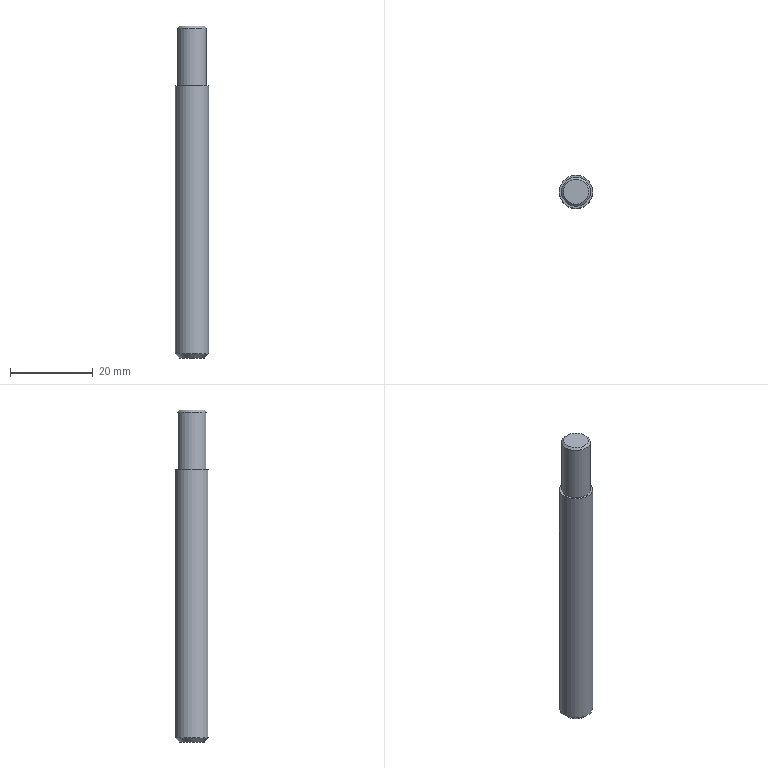Component | NX | LG_ADJ_SUPPORT_2 | 1 solid | 7 faces | box 8 x 8 x 80 mm | volume 3834 mm3 | plane 3 | cylinder 2 | cone 2 | commonest cylinder face diameters 8 x1 6.98 x1
STEP:
#1=CARTESIAN_POINT('',(0.,0.,0.));
#2=DIRECTION('',(0.,0.,1.));
#3=DIRECTION('',(1.,0.,0.));
#4=AXIS2_PLACEMENT_3D('',#1,#2,#3);
#5=CARTESIAN_POINT('',(-91.,-45.,-251.));
#6=VERTEX_POINT('',#5);
#7=CARTESIAN_POINT('',(-88.,-45.,-251.));
#8=DIRECTION('',(0.,0.,-1.));
#9=DIRECTION('',(-1.,0.,0.));
#10=AXIS2_PLACEMENT_3D('',#7,#8,#9);
#11=CIRCLE('',#10,3.);
#12=CARTESIAN_POINT('',(-88.,-45.,-251.));
#13=DIRECTION('',(0.,0.,-1.));
#14=DIRECTION('',(-1.,0.,0.));
#15=AXIS2_PLACEMENT_3D('',#12,#13,#14);
#16=PLANE('',#15);
#17=CARTESIAN_POINT('',(0.,0.));
#18=DIRECTION('',(1.,0.));
#19=AXIS2_PLACEMENT_2D('',#17,#18);
#20=CIRCLE('',#19,3.);
#21=(GEOMETRIC_REPRESENTATION_CONTEXT(2)PARAMETRIC_REPRESENTATION_CONTEXT()REPRESENTATION_CONTEXT('',''));
#22=DEFINITIONAL_REPRESENTATION('',(#20),#21);
#23=PCURVE('',#16,#22);
#24=CARTESIAN_POINT('',(-88.,-45.,-250.));
#25=DIRECTION('',(0.,0.,1.));
#26=DIRECTION('',(1.,0.,0.));
#27=AXIS2_PLACEMENT_3D('',#24,#25,#26);
#28=CONICAL_SURFACE('',#27,4.,0.7854);
#29=CARTESIAN_POINT('',(9.425,-1.));
#30=DIRECTION('',(-1.,0.));
#31=VECTOR('',#30,1.);
#32=LINE('',#29,#31);
#33=(GEOMETRIC_REPRESENTATION_CONTEXT(2)PARAMETRIC_REPRESENTATION_CONTEXT()REPRESENTATION_CONTEXT('',''));
#34=DEFINITIONAL_REPRESENTATION('',(#32),#33);
#35=PCURVE('',#28,#34);
#36=SURFACE_CURVE('',#11,(#23,#35),.PCURVE_S1.);
#37=EDGE_CURVE('',#6,#6,#36,.T.);
#38=ORIENTED_EDGE('',*,*,#37,.T.);
#39=EDGE_LOOP('',(#38));
#40=FACE_BOUND('',#39,.T.);
#41=ADVANCED_FACE('',(#40),#16,.T.);
#42=CARTESIAN_POINT('',(-92.,-45.,-185.4));
#43=VERTEX_POINT('',#42);
#44=CARTESIAN_POINT('',(-88.,-45.,-185.4));
#45=DIRECTION('',(0.,0.,1.));
#46=DIRECTION('',(-1.,0.,0.));
#47=AXIS2_PLACEMENT_3D('',#44,#45,#46);
#48=CIRCLE('',#47,4.);
#49=CARTESIAN_POINT('',(-88.,-45.,-251.));
#50=DIRECTION('',(0.,0.,1.));
#51=DIRECTION('',(1.,0.,0.));
#52=AXIS2_PLACEMENT_3D('',#49,#50,#51);
#53=CYLINDRICAL_SURFACE('',#52,4.);
#54=CARTESIAN_POINT('',(3.142,65.6));
#55=DIRECTION('',(1.,0.));
#56=VECTOR('',#55,1.);
#57=LINE('',#54,#56);
#58=(GEOMETRIC_REPRESENTATION_CONTEXT(2)PARAMETRIC_REPRESENTATION_CONTEXT()REPRESENTATION_CONTEXT('',''));
#59=DEFINITIONAL_REPRESENTATION('',(#57),#58);
#60=PCURVE('',#53,#59);
#61=CARTESIAN_POINT('',(-88.,-45.,-185.4));
#62=DIRECTION('',(0.,0.,-1.));
#63=DIRECTION('',(-1.,0.,0.));
#64=AXIS2_PLACEMENT_3D('',#61,#62,#63);
#65=PLANE('',#64);
#66=CARTESIAN_POINT('',(4.,0.));
#67=CARTESIAN_POINT('',(4.,-6.928));
#68=CARTESIAN_POINT('',(-2.,-3.464));
#69=CARTESIAN_POINT('',(-8.,-0.));
#70=CARTESIAN_POINT('',(-2.,3.464));
#71=CARTESIAN_POINT('',(4.,6.928));
#72=CARTESIAN_POINT('',(4.,0.));
#73=(BOUNDED_CURVE()B_SPLINE_CURVE(2,(#66,#67,#68,#69,#70,#71,#72),.UNSPECIFIED.,.T.,.F.)B_SPLINE_CURVE_WITH_KNOTS((1,2,2,2,2,1),(-2.094,0.,2.094,4.189,6.283,8.378),.UNSPECIFIED.)CURVE()GEOMETRIC_REPRESENTATION_ITEM()RATIONAL_B_SPLINE_CURVE((1.,0.5,1.,0.5,1.,0.5,1.))REPRESENTATION_ITEM(''));
#74=(GEOMETRIC_REPRESENTATION_CONTEXT(2)PARAMETRIC_REPRESENTATION_CONTEXT()REPRESENTATION_CONTEXT('',''));
#75=DEFINITIONAL_REPRESENTATION('',(#73),#74);
#76=PCURVE('',#65,#75);
#77=SURFACE_CURVE('',#48,(#60,#76),.PCURVE_S1.);
#78=EDGE_CURVE('',#43,#43,#77,.T.);
#79=ORIENTED_EDGE('',*,*,#78,.F.);
#80=CARTESIAN_POINT('',(-92.,-45.,-250.));
#81=VERTEX_POINT('',#80);
#82=CARTESIAN_POINT('',(-92.,-45.,-250.));
#83=CARTESIAN_POINT('',(-92.,-45.,-185.4));
#84=B_SPLINE_CURVE_WITH_KNOTS('',1,(#82,#83),.UNSPECIFIED.,.F.,.F.,(2,2),(1.,65.6),.PIECEWISE_BEZIER_KNOTS.);
#85=CARTESIAN_POINT('',(3.142,0.));
#86=DIRECTION('',(0.,1.));
#87=VECTOR('',#86,1.);
#88=LINE('',#85,#87);
#89=(GEOMETRIC_REPRESENTATION_CONTEXT(2)PARAMETRIC_REPRESENTATION_CONTEXT()REPRESENTATION_CONTEXT('',''));
#90=DEFINITIONAL_REPRESENTATION('',(#88),#89);
#91=PCURVE('',#53,#90);
#92=CARTESIAN_POINT('',(9.425,0.));
#93=DIRECTION('',(0.,1.));
#94=VECTOR('',#93,1.);
#95=LINE('',#92,#94);
#96=(GEOMETRIC_REPRESENTATION_CONTEXT(2)PARAMETRIC_REPRESENTATION_CONTEXT()REPRESENTATION_CONTEXT('',''));
#97=DEFINITIONAL_REPRESENTATION('',(#95),#96);
#98=PCURVE('',#53,#97);
#99=SEAM_CURVE('',#84,(#91,#98),.PCURVE_S1.);
#100=EDGE_CURVE('',#81,#43,#99,.T.);
#101=ORIENTED_EDGE('',*,*,#100,.F.);
#102=CARTESIAN_POINT('',(-88.,-45.,-250.));
#103=DIRECTION('',(0.,0.,1.));
#104=DIRECTION('',(-1.,0.,0.));
#105=AXIS2_PLACEMENT_3D('',#102,#103,#104);
#106=CIRCLE('',#105,4.);
#107=CARTESIAN_POINT('',(3.142,1.));
#108=DIRECTION('',(1.,0.));
#109=VECTOR('',#108,1.);
#110=LINE('',#107,#109);
#111=(GEOMETRIC_REPRESENTATION_CONTEXT(2)PARAMETRIC_REPRESENTATION_CONTEXT()REPRESENTATION_CONTEXT('',''));
#112=DEFINITIONAL_REPRESENTATION('',(#110),#111);
#113=PCURVE('',#53,#112);
#114=CARTESIAN_POINT('',(3.142,0.));
#115=DIRECTION('',(1.,0.));
#116=VECTOR('',#115,1.);
#117=LINE('',#114,#116);
#118=(GEOMETRIC_REPRESENTATION_CONTEXT(2)PARAMETRIC_REPRESENTATION_CONTEXT()REPRESENTATION_CONTEXT('',''));
#119=DEFINITIONAL_REPRESENTATION('',(#117),#118);
#120=PCURVE('',#28,#119);
#121=SURFACE_CURVE('',#106,(#113,#120),.PCURVE_S1.);
#122=EDGE_CURVE('',#81,#81,#121,.T.);
#123=ORIENTED_EDGE('',*,*,#122,.T.);
#124=ORIENTED_EDGE('',*,*,#100,.T.);
#125=EDGE_LOOP('',(#79,#101,#123,#124));
#126=FACE_BOUND('',#125,.T.);
#127=ADVANCED_FACE('',(#126),#53,.T.);
#128=ORIENTED_EDGE('',*,*,#37,.F.);
#129=CARTESIAN_POINT('',(-91.,-45.,-251.));
#130=CARTESIAN_POINT('',(-92.,-45.,-250.));
#131=B_SPLINE_CURVE_WITH_KNOTS('',1,(#129,#130),.UNSPECIFIED.,.F.,.F.,(2,2),(-1.414,0.),.PIECEWISE_BEZIER_KNOTS.);
#132=CARTESIAN_POINT('',(9.425,0.));
#133=DIRECTION('',(0.,1.));
#134=VECTOR('',#133,1.);
#135=LINE('',#132,#134);
#136=(GEOMETRIC_REPRESENTATION_CONTEXT(2)PARAMETRIC_REPRESENTATION_CONTEXT()REPRESENTATION_CONTEXT('',''));
#137=DEFINITIONAL_REPRESENTATION('',(#135),#136);
#138=PCURVE('',#28,#137);
#139=CARTESIAN_POINT('',(3.142,0.));
#140=DIRECTION('',(0.,1.));
#141=VECTOR('',#140,1.);
#142=LINE('',#139,#141);
#143=(GEOMETRIC_REPRESENTATION_CONTEXT(2)PARAMETRIC_REPRESENTATION_CONTEXT()REPRESENTATION_CONTEXT('',''));
#144=DEFINITIONAL_REPRESENTATION('',(#142),#143);
#145=PCURVE('',#28,#144);
#146=SEAM_CURVE('',#131,(#138,#145),.PCURVE_S1.);
#147=EDGE_CURVE('',#6,#81,#146,.T.);
#148=ORIENTED_EDGE('',*,*,#147,.T.);
#149=ORIENTED_EDGE('',*,*,#122,.F.);
#150=ORIENTED_EDGE('',*,*,#147,.F.);
#151=EDGE_LOOP('',(#128,#148,#149,#150));
#152=FACE_BOUND('',#151,.T.);
#153=ADVANCED_FACE('',(#152),#28,.T.);
#154=ORIENTED_EDGE('',*,*,#78,.T.);
#155=EDGE_LOOP('',(#154));
#156=FACE_BOUND('',#155,.T.);
#157=CARTESIAN_POINT('',(-91.49,-45.,-185.4));
#158=VERTEX_POINT('',#157);
#159=CARTESIAN_POINT('',(-88.,-45.,-185.4));
#160=DIRECTION('',(0.,0.,1.));
#161=DIRECTION('',(-1.,0.,0.));
#162=AXIS2_PLACEMENT_3D('',#159,#160,#161);
#163=CIRCLE('',#162,3.49);
#164=CARTESIAN_POINT('',(3.49,0.));
#165=CARTESIAN_POINT('',(3.49,-6.045));
#166=CARTESIAN_POINT('',(-1.745,-3.022));
#167=CARTESIAN_POINT('',(-6.98,-0.));
#168=CARTESIAN_POINT('',(-1.745,3.022));
#169=CARTESIAN_POINT('',(3.49,6.045));
#170=CARTESIAN_POINT('',(3.49,0.));
#171=(BOUNDED_CURVE()B_SPLINE_CURVE(2,(#164,#165,#166,#167,#168,#169,#170),.UNSPECIFIED.,.T.,.F.)B_SPLINE_CURVE_WITH_KNOTS((1,2,2,2,2,1),(-2.094,0.,2.094,4.189,6.283,8.378),.UNSPECIFIED.)CURVE()GEOMETRIC_REPRESENTATION_ITEM()RATIONAL_B_SPLINE_CURVE((1.,0.5,1.,0.5,1.,0.5,1.))REPRESENTATION_ITEM(''));
#172=(GEOMETRIC_REPRESENTATION_CONTEXT(2)PARAMETRIC_REPRESENTATION_CONTEXT()REPRESENTATION_CONTEXT('',''));
#173=DEFINITIONAL_REPRESENTATION('',(#171),#172);
#174=PCURVE('',#65,#173);
#175=CARTESIAN_POINT('',(-88.,-45.,-186.4));
#176=DIRECTION('',(0.,0.,1.));
#177=DIRECTION('',(1.,0.,0.));
#178=AXIS2_PLACEMENT_3D('',#175,#176,#177);
#179=CYLINDRICAL_SURFACE('',#178,3.49);
#180=CARTESIAN_POINT('',(3.142,1.));
#181=DIRECTION('',(1.,0.));
#182=VECTOR('',#181,1.);
#183=LINE('',#180,#182);
#184=(GEOMETRIC_REPRESENTATION_CONTEXT(2)PARAMETRIC_REPRESENTATION_CONTEXT()REPRESENTATION_CONTEXT('',''));
#185=DEFINITIONAL_REPRESENTATION('',(#183),#184);
#186=PCURVE('',#179,#185);
#187=SURFACE_CURVE('',#163,(#174,#186),.PCURVE_S1.);
#188=EDGE_CURVE('',#158,#158,#187,.T.);
#189=ORIENTED_EDGE('',*,*,#188,.F.);
#190=EDGE_LOOP('',(#189));
#191=FACE_BOUND('',#190,.T.);
#192=ADVANCED_FACE('',(#156,#191),#65,.F.);
#193=CARTESIAN_POINT('',(-91.49,-45.,-171.49));
#194=VERTEX_POINT('',#193);
#195=CARTESIAN_POINT('',(-88.,-45.,-171.49));
#196=DIRECTION('',(0.,0.,1.));
#197=DIRECTION('',(-1.,0.,0.));
#198=AXIS2_PLACEMENT_3D('',#195,#196,#197);
#199=CIRCLE('',#198,3.49);
#200=CARTESIAN_POINT('',(3.142,14.91));
#201=DIRECTION('',(1.,0.));
#202=VECTOR('',#201,1.);
#203=LINE('',#200,#202);
#204=(GEOMETRIC_REPRESENTATION_CONTEXT(2)PARAMETRIC_REPRESENTATION_CONTEXT()REPRESENTATION_CONTEXT('',''));
#205=DEFINITIONAL_REPRESENTATION('',(#203),#204);
#206=PCURVE('',#179,#205);
#207=CARTESIAN_POINT('',(-88.,-45.,-172.));
#208=DIRECTION('',(0.,0.,-1.));
#209=DIRECTION('',(-1.,0.,0.));
#210=AXIS2_PLACEMENT_3D('',#207,#208,#209);
#211=CONICAL_SURFACE('',#210,4.,0.7854);
#212=CARTESIAN_POINT('',(6.283,-0.51));
#213=DIRECTION('',(-1.,0.));
#214=VECTOR('',#213,1.);
#215=LINE('',#212,#214);
#216=(GEOMETRIC_REPRESENTATION_CONTEXT(2)PARAMETRIC_REPRESENTATION_CONTEXT()REPRESENTATION_CONTEXT('',''));
#217=DEFINITIONAL_REPRESENTATION('',(#215),#216);
#218=PCURVE('',#211,#217);
#219=SURFACE_CURVE('',#199,(#206,#218),.PCURVE_S1.);
#220=EDGE_CURVE('',#194,#194,#219,.T.);
#221=ORIENTED_EDGE('',*,*,#220,.F.);
#222=CARTESIAN_POINT('',(-91.49,-45.,-185.4));
#223=CARTESIAN_POINT('',(-91.49,-45.,-171.49));
#224=B_SPLINE_CURVE_WITH_KNOTS('',1,(#222,#223),.UNSPECIFIED.,.F.,.F.,(2,2),(1.,14.91),.PIECEWISE_BEZIER_KNOTS.);
#225=CARTESIAN_POINT('',(3.142,0.));
#226=DIRECTION('',(0.,1.));
#227=VECTOR('',#226,1.);
#228=LINE('',#225,#227);
#229=(GEOMETRIC_REPRESENTATION_CONTEXT(2)PARAMETRIC_REPRESENTATION_CONTEXT()REPRESENTATION_CONTEXT('',''));
#230=DEFINITIONAL_REPRESENTATION('',(#228),#229);
#231=PCURVE('',#179,#230);
#232=CARTESIAN_POINT('',(9.425,0.));
#233=DIRECTION('',(0.,1.));
#234=VECTOR('',#233,1.);
#235=LINE('',#232,#234);
#236=(GEOMETRIC_REPRESENTATION_CONTEXT(2)PARAMETRIC_REPRESENTATION_CONTEXT()REPRESENTATION_CONTEXT('',''));
#237=DEFINITIONAL_REPRESENTATION('',(#235),#236);
#238=PCURVE('',#179,#237);
#239=SEAM_CURVE('',#224,(#231,#238),.PCURVE_S1.);
#240=EDGE_CURVE('',#158,#194,#239,.T.);
#241=ORIENTED_EDGE('',*,*,#240,.F.);
#242=ORIENTED_EDGE('',*,*,#188,.T.);
#243=ORIENTED_EDGE('',*,*,#240,.T.);
#244=EDGE_LOOP('',(#221,#241,#242,#243));
#245=FACE_BOUND('',#244,.T.);
#246=ADVANCED_FACE('',(#245),#179,.T.);
#247=CARTESIAN_POINT('',(-85.,-45.,-171.));
#248=VERTEX_POINT('',#247);
#249=CARTESIAN_POINT('',(-91.,-45.,-171.));
#250=VERTEX_POINT('',#249);
#251=CARTESIAN_POINT('',(-88.,-45.,-171.));
#252=DIRECTION('',(0.,0.,1.));
#253=DIRECTION('',(1.,0.,0.));
#254=AXIS2_PLACEMENT_3D('',#251,#252,#253);
#255=CIRCLE('',#254,3.);
#256=CARTESIAN_POINT('',(-88.,-45.,-171.));
#257=DIRECTION('',(0.,0.,1.));
#258=DIRECTION('',(1.,0.,0.));
#259=AXIS2_PLACEMENT_3D('',#256,#257,#258);
#260=PLANE('',#259);
#261=CARTESIAN_POINT('',(0.,0.));
#262=DIRECTION('',(1.,0.));
#263=AXIS2_PLACEMENT_2D('',#261,#262);
#264=CIRCLE('',#263,3.);
#265=(GEOMETRIC_REPRESENTATION_CONTEXT(2)PARAMETRIC_REPRESENTATION_CONTEXT()REPRESENTATION_CONTEXT('',''));
#266=DEFINITIONAL_REPRESENTATION('',(#264),#265);
#267=PCURVE('',#260,#266);
#268=CARTESIAN_POINT('',(3.142,-1.));
#269=DIRECTION('',(-1.,0.));
#270=VECTOR('',#269,1.);
#271=LINE('',#268,#270);
#272=(GEOMETRIC_REPRESENTATION_CONTEXT(2)PARAMETRIC_REPRESENTATION_CONTEXT()REPRESENTATION_CONTEXT('',''));
#273=DEFINITIONAL_REPRESENTATION('',(#271),#272);
#274=PCURVE('',#211,#273);
#275=SURFACE_CURVE('',#255,(#267,#274),.PCURVE_S1.);
#276=EDGE_CURVE('',#248,#250,#275,.T.);
#277=ORIENTED_EDGE('',*,*,#276,.T.);
#278=CARTESIAN_POINT('',(-88.,-45.,-171.));
#279=DIRECTION('',(0.,0.,1.));
#280=DIRECTION('',(1.,0.,0.));
#281=AXIS2_PLACEMENT_3D('',#278,#279,#280);
#282=CIRCLE('',#281,3.);
#283=CARTESIAN_POINT('',(0.,0.));
#284=DIRECTION('',(1.,0.));
#285=AXIS2_PLACEMENT_2D('',#283,#284);
#286=CIRCLE('',#285,3.);
#287=(GEOMETRIC_REPRESENTATION_CONTEXT(2)PARAMETRIC_REPRESENTATION_CONTEXT()REPRESENTATION_CONTEXT('',''));
#288=DEFINITIONAL_REPRESENTATION('',(#286),#287);
#289=PCURVE('',#260,#288);
#290=CARTESIAN_POINT('',(9.425,-1.));
#291=DIRECTION('',(-1.,0.));
#292=VECTOR('',#291,1.);
#293=LINE('',#290,#292);
#294=(GEOMETRIC_REPRESENTATION_CONTEXT(2)PARAMETRIC_REPRESENTATION_CONTEXT()REPRESENTATION_CONTEXT('',''));
#295=DEFINITIONAL_REPRESENTATION('',(#293),#294);
#296=PCURVE('',#211,#295);
#297=SURFACE_CURVE('',#282,(#289,#296),.PCURVE_S1.);
#298=EDGE_CURVE('',#250,#248,#297,.T.);
#299=ORIENTED_EDGE('',*,*,#298,.T.);
#300=EDGE_LOOP('',(#277,#299));
#301=FACE_BOUND('',#300,.T.);
#302=ADVANCED_FACE('',(#301),#260,.T.);
#303=ORIENTED_EDGE('',*,*,#298,.F.);
#304=CARTESIAN_POINT('',(-91.,-45.,-171.));
#305=CARTESIAN_POINT('',(-91.49,-45.,-171.49));
#306=B_SPLINE_CURVE_WITH_KNOTS('',1,(#304,#305),.UNSPECIFIED.,.F.,.F.,(2,2),(-1.414,-0.7212),.PIECEWISE_BEZIER_KNOTS.);
#307=CARTESIAN_POINT('',(6.283,0.));
#308=DIRECTION('',(0.,1.));
#309=VECTOR('',#308,1.);
#310=LINE('',#307,#309);
#311=(GEOMETRIC_REPRESENTATION_CONTEXT(2)PARAMETRIC_REPRESENTATION_CONTEXT()REPRESENTATION_CONTEXT('',''));
#312=DEFINITIONAL_REPRESENTATION('',(#310),#311);
#313=PCURVE('',#211,#312);
#314=CARTESIAN_POINT('',(0.,0.));
#315=DIRECTION('',(0.,1.));
#316=VECTOR('',#315,1.);
#317=LINE('',#314,#316);
#318=(GEOMETRIC_REPRESENTATION_CONTEXT(2)PARAMETRIC_REPRESENTATION_CONTEXT()REPRESENTATION_CONTEXT('',''));
#319=DEFINITIONAL_REPRESENTATION('',(#317),#318);
#320=PCURVE('',#211,#319);
#321=SEAM_CURVE('',#306,(#313,#320),.PCURVE_S1.);
#322=EDGE_CURVE('',#250,#194,#321,.T.);
#323=ORIENTED_EDGE('',*,*,#322,.T.);
#324=ORIENTED_EDGE('',*,*,#220,.T.);
#325=ORIENTED_EDGE('',*,*,#322,.F.);
#326=ORIENTED_EDGE('',*,*,#276,.F.);
#327=EDGE_LOOP('',(#303,#323,#324,#325,#326));
#328=FACE_BOUND('',#327,.T.);
#329=ADVANCED_FACE('',(#328),#211,.T.);
#330=CLOSED_SHELL('',(#41,#127,#153,#192,#246,#302,#329));
#331=MANIFOLD_SOLID_BREP('',#330);
#332=(LENGTH_UNIT()NAMED_UNIT(*)SI_UNIT(.MILLI.,.METRE.));
#333=UNCERTAINTY_MEASURE_WITH_UNIT(LENGTH_MEASURE(0.000005),#332,'','');
#334=(NAMED_UNIT(*)PLANE_ANGLE_UNIT()SI_UNIT($,.RADIAN.));
#335=(NAMED_UNIT(*)SI_UNIT($,.STERADIAN.)SOLID_ANGLE_UNIT());
#336=(GEOMETRIC_REPRESENTATION_CONTEXT(3)GLOBAL_UNCERTAINTY_ASSIGNED_CONTEXT((#333))GLOBAL_UNIT_ASSIGNED_CONTEXT((#332,#334,#335))REPRESENTATION_CONTEXT('',''));
#337=ADVANCED_BREP_SHAPE_REPRESENTATION('',(#4,#331),#336);